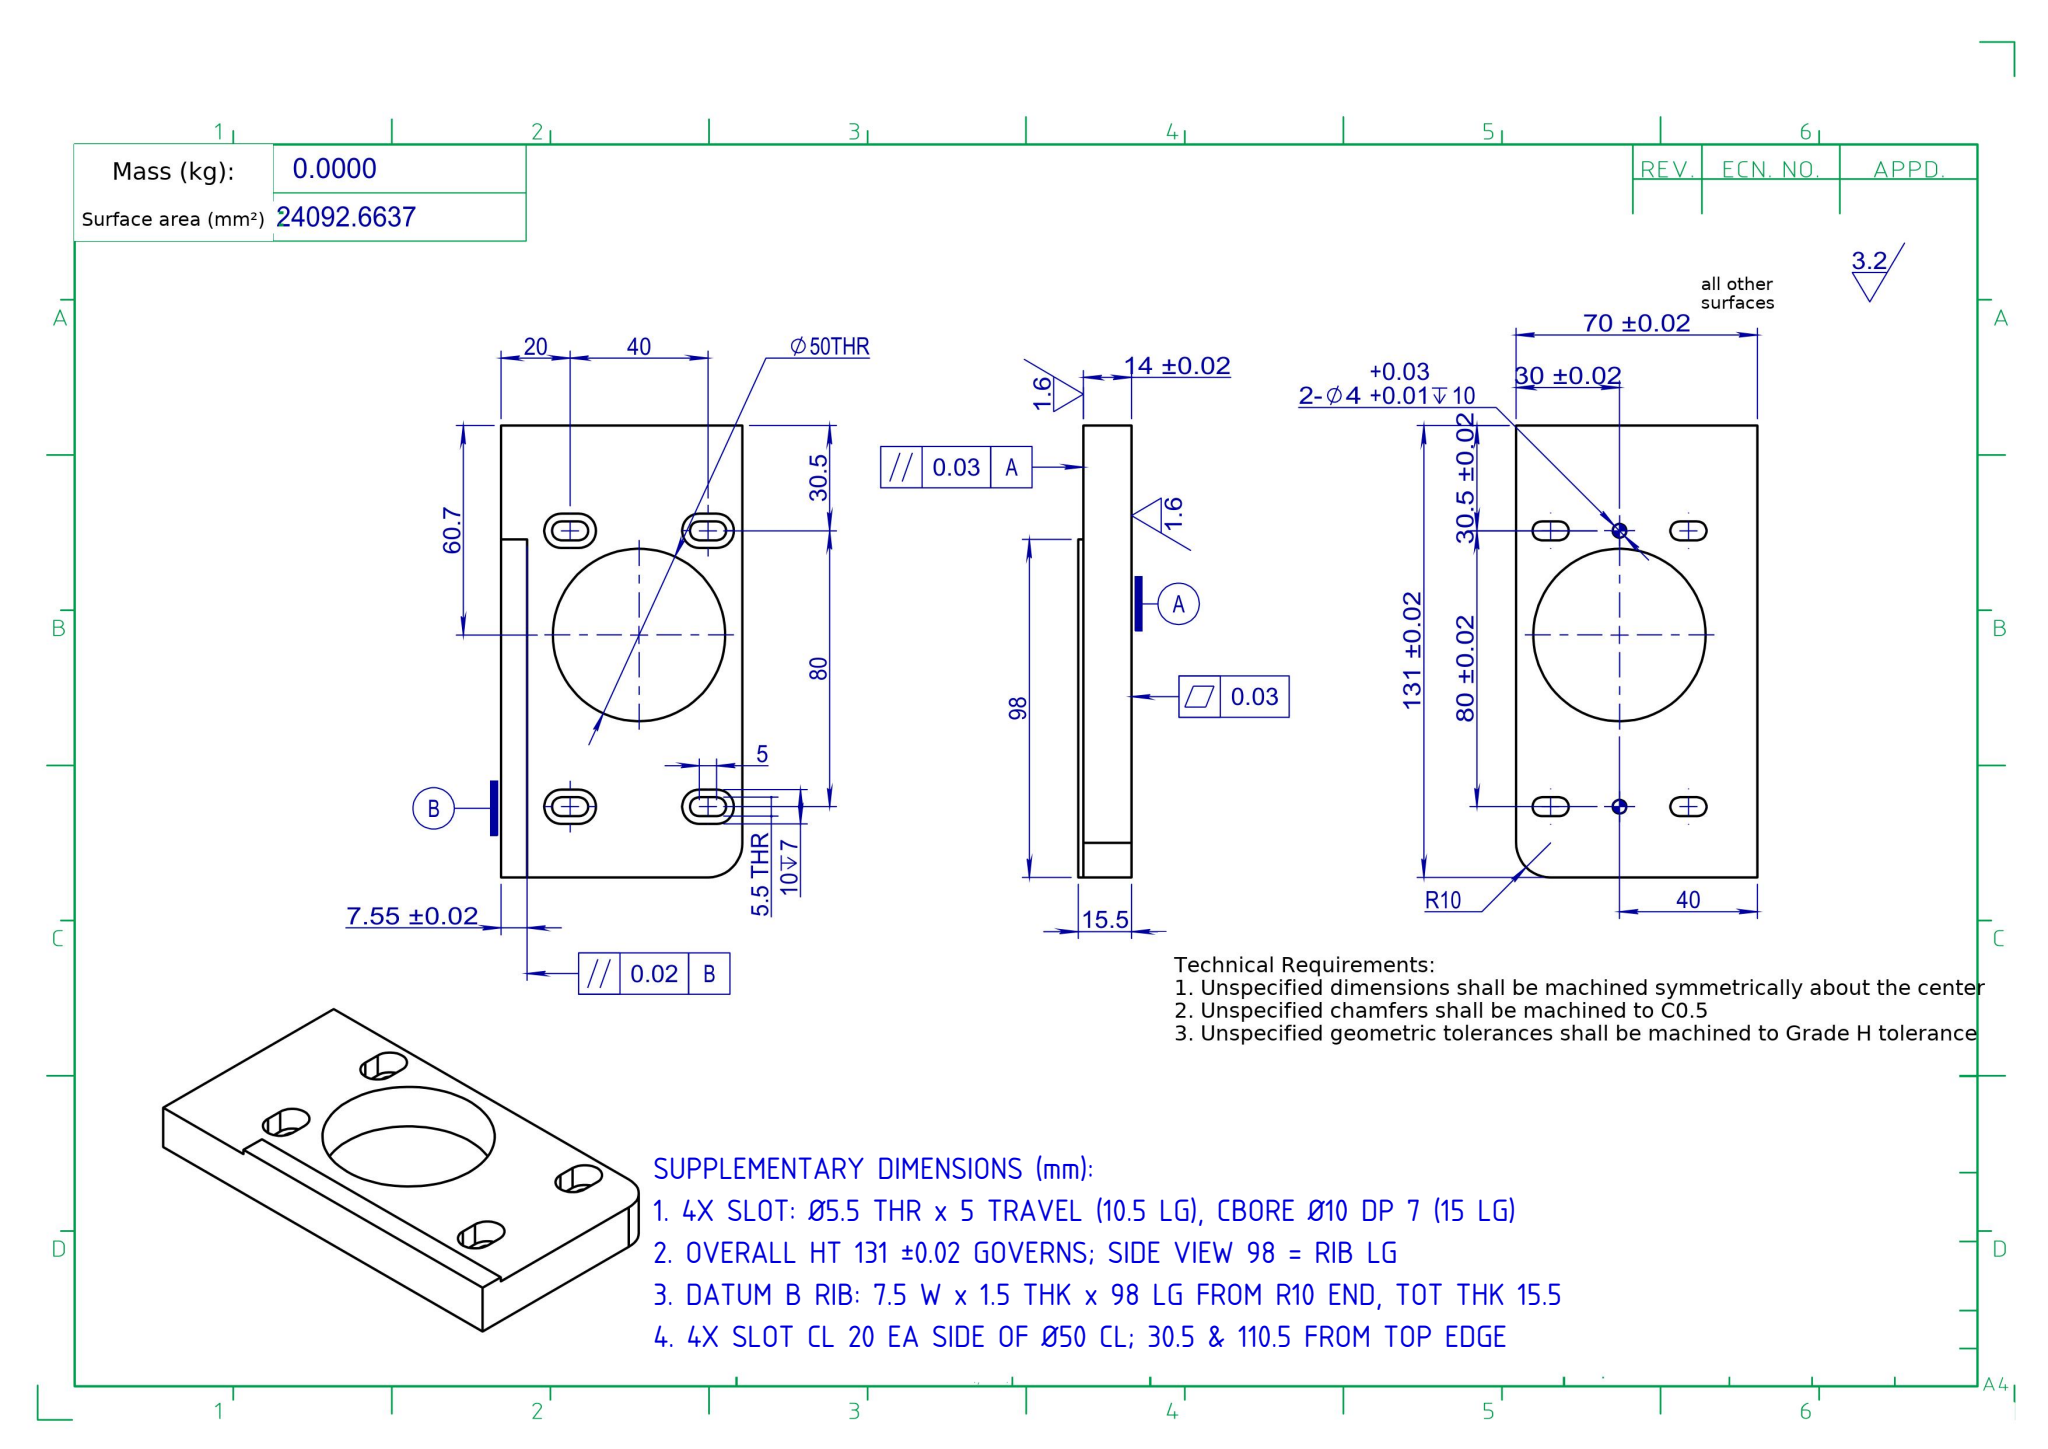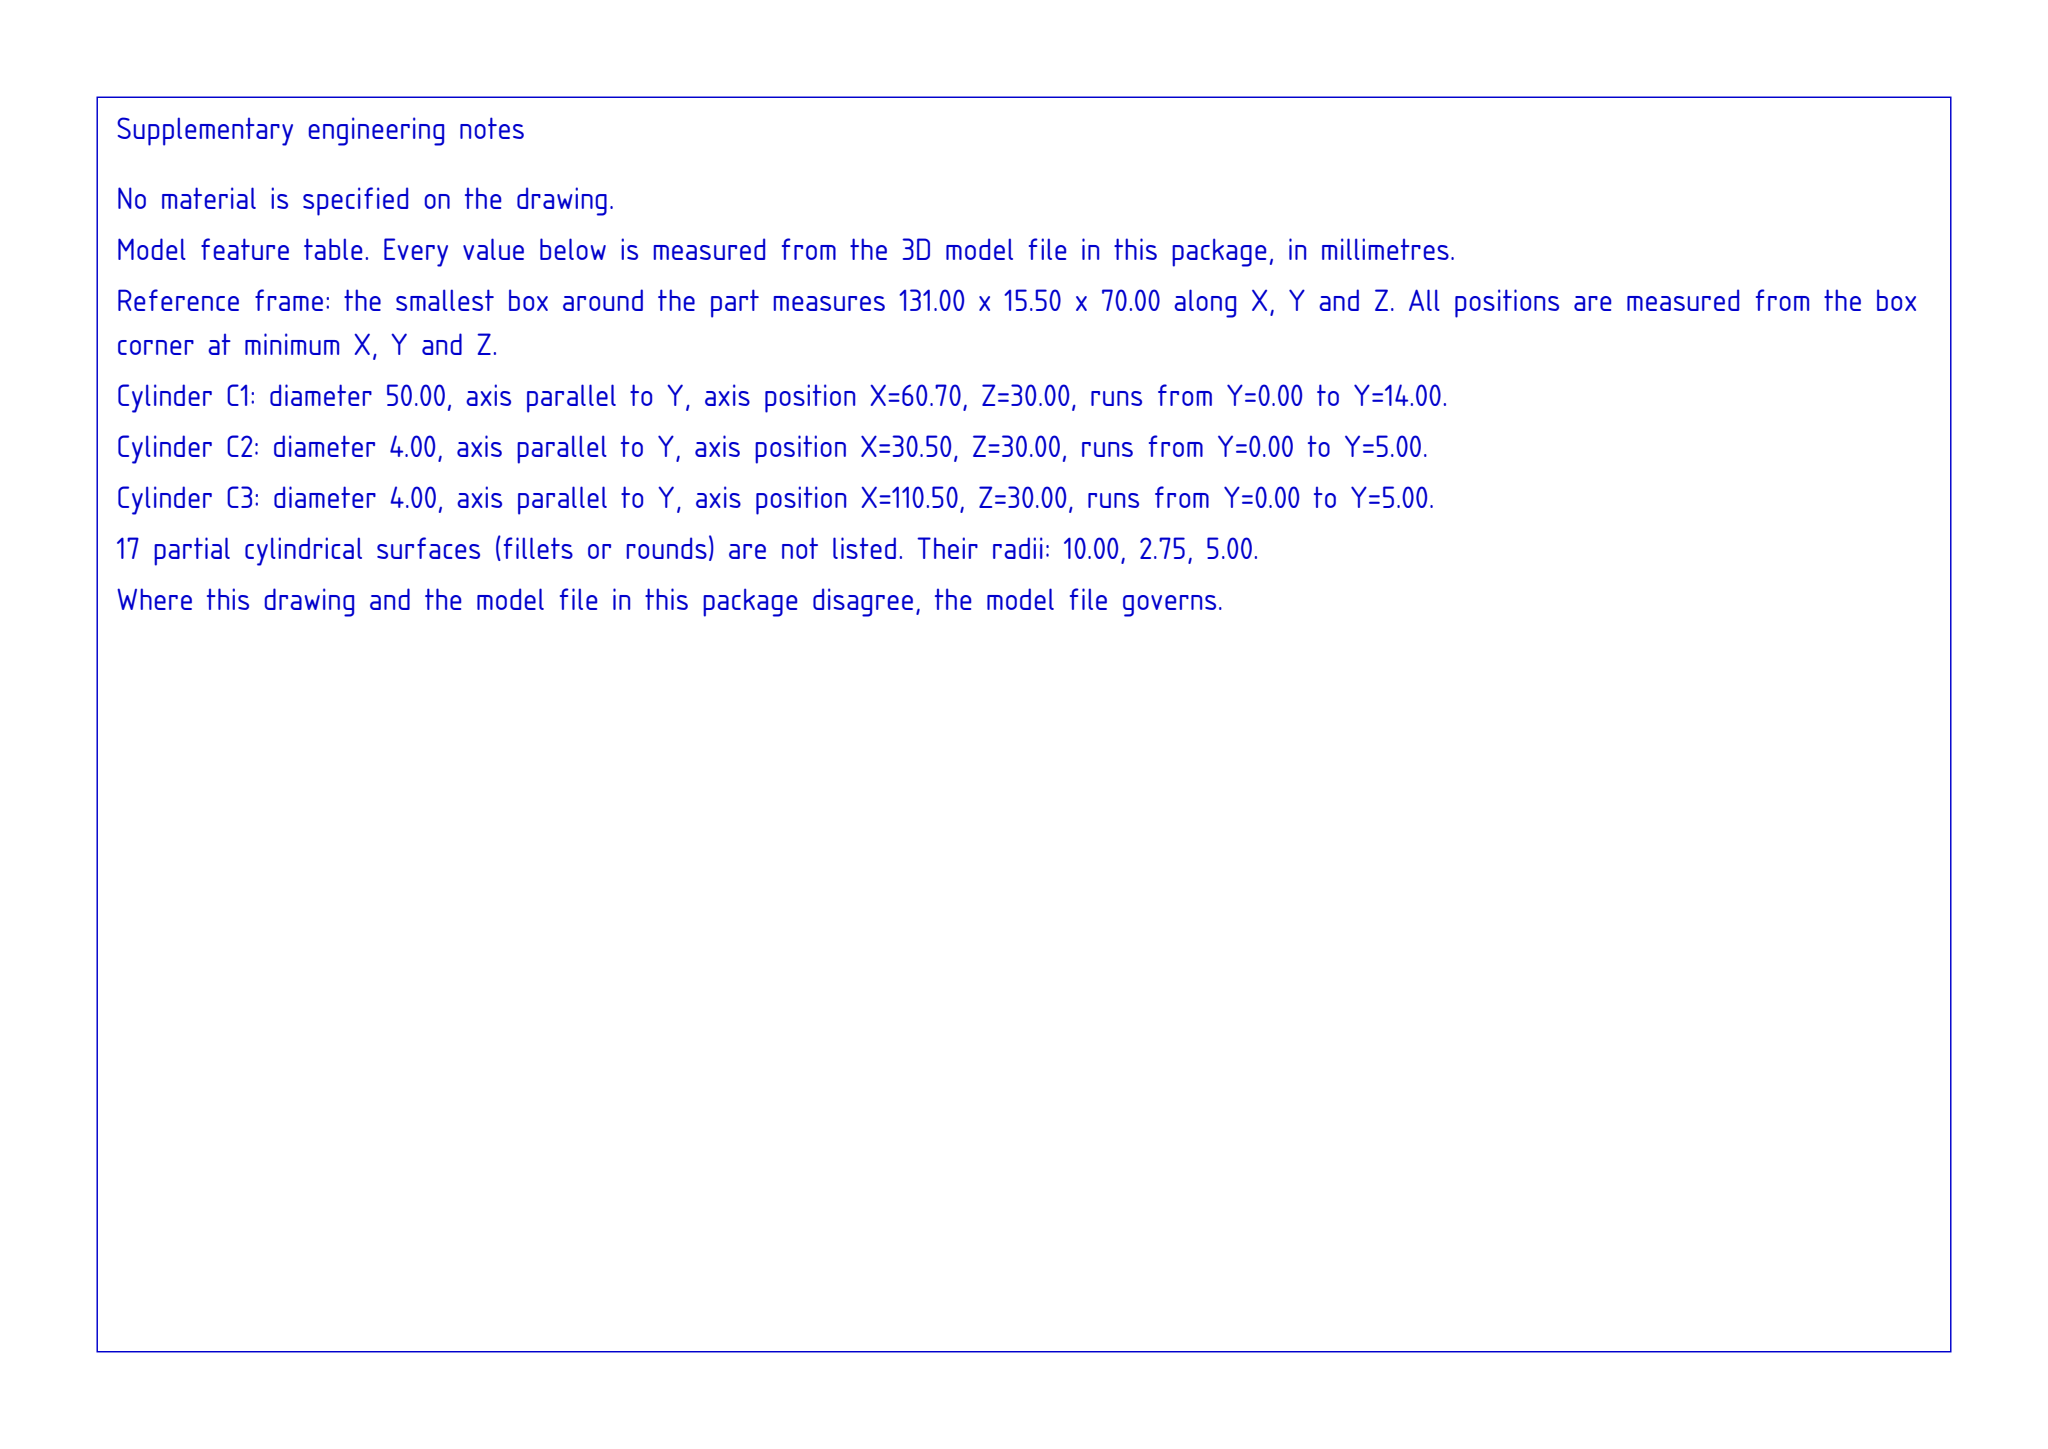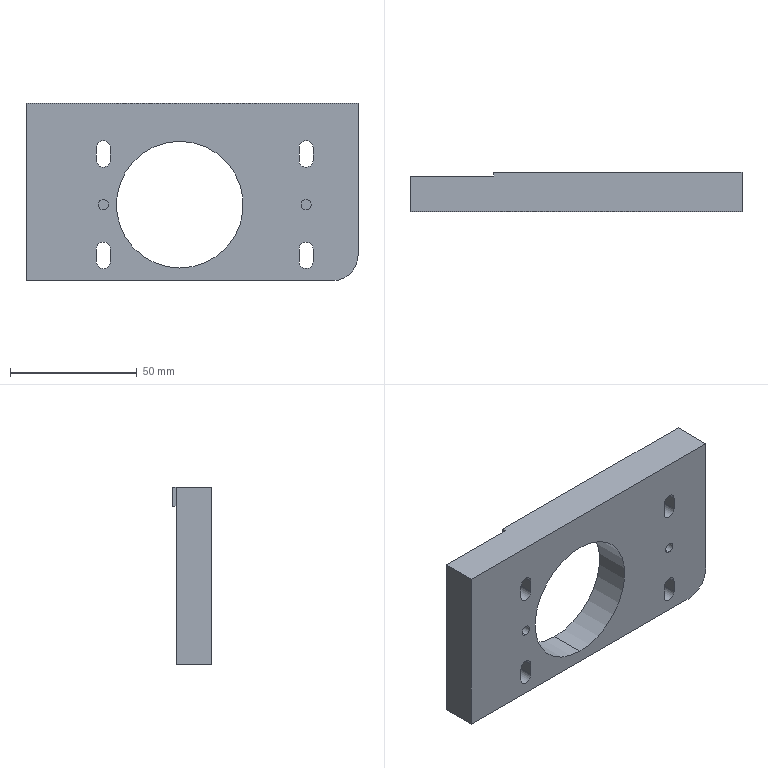Part | SolidWorks | mm | 1 solid | 62 faces | box 131 x 15.5 x 70 mm | volume 96533 mm3 | cylinder 31 | plane 31 | commonest cylinder face diameters 10 x12 5.5 x12 4 x4 50 x2 20 x1
build123d program:
from build123d import *

# Parameters (mm, degrees)
SKETCH1_W           = 131
SKETCH1_H           = 70
BOSS_EXTRUDE1_DEPTH = 18
CUT_EXTRUDE1_REACH  = 138.785
SKETCH2_W           = 62.5
SKETCH2_H           = 4
CUT_EXTRUDE2_REACH  = 99.541
SKETCH3_W           = 33
SKETCH3_H           = 4
SKETCH5_R           = 25
CUT_EXTRUDE4_DEPTH  = 76.573
CUT_EXTRUDE5_DEPTH  = 76.573
CUT_EXTRUDE6_DEPTH  = 7
SKETCH10_R          = 2
CUT_EXTRUDE7_DEPTH  = 5
FILLET1_R           = 10
SKETCH12_W          = 98
SKETCH12_H          = 7.5
CUT_EXTRUDE8_DEPTH  = 2.5


with BuildPart() as part:
    # Sketch1 → Boss-Extrude1 (new body)
    with BuildSketch(Plane(origin=(0, 0, 0), x_dir=(1, 0, 0), z_dir=(0, 1, 0))):
        Rectangle(SKETCH1_W, SKETCH1_H)
    extrude(amount=BOSS_EXTRUDE1_DEPTH)

    # Sketch2 → Cut-Extrude1 (cut, up to next)
    with BuildSketch(Plane(origin=(65.5, 0, 0), x_dir=(0, 0, -1), z_dir=(1, 0, 0)), mode=Mode.PRIVATE) as cut_extrude1_sk1:
        with Locations((3.75, 16)):
            Rectangle(SKETCH2_W, SKETCH2_H)
    cut_extrude1_tool1 = extrude(cut_extrude1_sk1.sketch, amount=-CUT_EXTRUDE1_REACH, mode=Mode.PRIVATE) & part.part
    add(cut_extrude1_tool1.solids().sort_by_distance((65.5, 16, -3.75))[0], mode=Mode.SUBTRACT)

    # Sketch3 → Cut-Extrude2 (cut, up to next)
    with BuildSketch(Plane.XY.offset(35), mode=Mode.PRIVATE) as cut_extrude2_sk1:
        with Locations((-49, 16)):
            Rectangle(SKETCH3_W, SKETCH3_H)
    cut_extrude2_tool1 = extrude(cut_extrude2_sk1.sketch, amount=-CUT_EXTRUDE2_REACH, mode=Mode.PRIVATE) & part.part
    add(cut_extrude2_tool1.solids().sort_by_distance((-49, 16, 35))[0], mode=Mode.SUBTRACT)

    # Sketch5 → Cut-Extrude4 (cut, through all)
    with BuildSketch(Plane(origin=(0, 14, 0), x_dir=(1, 0, 0), z_dir=(0, 1, 0))):
        with Locations(Location((-4.8, 5, 0), (0, 0, 270))):
            Circle(SKETCH5_R)
    extrude(amount=-CUT_EXTRUDE4_DEPTH, mode=Mode.SUBTRACT)

    # Sketch6 → Cut-Extrude5 (cut, through all)
    with BuildSketch(Plane(origin=(0, 14, 0), x_dir=(1, 0, 0), z_dir=(0, 1, 0))):
        with BuildLine():
            Line((-37.75, -17.5), (-37.75, -12.5))
            ThreePointArc((-37.75, -12.5), (-35, -9.75), (-32.25, -12.5))
            Line((-32.25, -12.5), (-32.25, -17.5))
            ThreePointArc((-32.25, -17.5), (-35, -20.25), (-37.75, -17.5))
        make_face()
        with BuildLine():
            Line((42.25, -17.5), (42.25, -12.5))
            ThreePointArc((42.25, -12.5), (45, -9.75), (47.75, -12.5))
            Line((47.75, -12.5), (47.75, -17.5))
            ThreePointArc((47.75, -17.5), (45, -20.25), (42.25, -17.5))
        make_face()
        with BuildLine():
            Line((42.25, 22.5), (42.25, 27.5))
            ThreePointArc((42.25, 27.5), (45, 30.25), (47.75, 27.5))
            Line((47.75, 27.5), (47.75, 22.5))
            ThreePointArc((47.75, 22.5), (45, 19.75), (42.25, 22.5))
        make_face()
        with BuildLine():
            Line((-37.75, 22.5), (-37.75, 27.5))
            ThreePointArc((-37.75, 27.5), (-35, 30.25), (-32.25, 27.5))
            Line((-32.25, 27.5), (-32.25, 22.5))
            ThreePointArc((-32.25, 22.5), (-35, 19.75), (-37.75, 22.5))
        make_face()
    extrude(amount=-CUT_EXTRUDE5_DEPTH, mode=Mode.SUBTRACT)

    # Sketch9 → Cut-Extrude6 (cut)
    with BuildSketch(Plane(origin=(0, 14, 0), x_dir=(1, 0, 0), z_dir=(0, 1, 0))):
        with BuildLine():
            Line((-30, -12.5), (-30, -17.5))
            ThreePointArc((-30, -17.5), (-35, -22.5), (-40, -17.5))
            Line((-40, -17.5), (-40, -12.5))
            ThreePointArc((-40, -12.5), (-35, -7.5), (-30, -12.5))
        make_face()
        with BuildLine():
            Line((-30, 27.5), (-30, 22.5))
            ThreePointArc((-30, 22.5), (-35, 17.5), (-40, 22.5))
            Line((-40, 22.5), (-40, 27.5))
            ThreePointArc((-40, 27.5), (-35, 32.5), (-30, 27.5))
        make_face()
        with BuildLine():
            Line((50, 27.5), (50, 22.5))
            ThreePointArc((50, 22.5), (45, 17.5), (40, 22.5))
            Line((40, 22.5), (40, 27.5))
            ThreePointArc((40, 27.5), (45, 32.5), (50, 27.5))
        make_face()
        with BuildLine():
            Line((50, -12.5), (50, -17.5))
            ThreePointArc((50, -17.5), (45, -22.5), (40, -17.5))
            Line((40, -17.5), (40, -12.5))
            ThreePointArc((40, -12.5), (45, -7.5), (50, -12.5))
        make_face()
    extrude(amount=-CUT_EXTRUDE6_DEPTH, mode=Mode.SUBTRACT)

    # Sketch10 → Cut-Extrude7 (cut)
    with BuildSketch(Plane(origin=(0, 0, 0), x_dir=(1, 0, 0), z_dir=(0, 1, 0))):
        with Locations(Location((45, 5, 0), (0, 0, 270))):
            Circle(SKETCH10_R)
        with Locations(Location((-35, 5, 0), (0, 0, 270))):
            Circle(SKETCH10_R)
    extrude(amount=CUT_EXTRUDE7_DEPTH, mode=Mode.SUBTRACT)

    # Fillet1
    fillet1_edges = [part.edges().sort_by_distance(p)[0] for p in [
        (65.5, 7, -35),
    ]]
    fillet(fillet1_edges, radius=FILLET1_R)

    # Sketch12 → Cut-Extrude8 (cut)
    with BuildSketch(Plane(origin=(0, 18, 0), x_dir=(1, 0, 0), z_dir=(0, 1, 0))):
        with Locations((16.5, -31.25)):
            Rectangle(SKETCH12_W, SKETCH12_H)
    extrude(amount=-CUT_EXTRUDE8_DEPTH, mode=Mode.SUBTRACT)


solid = part.part